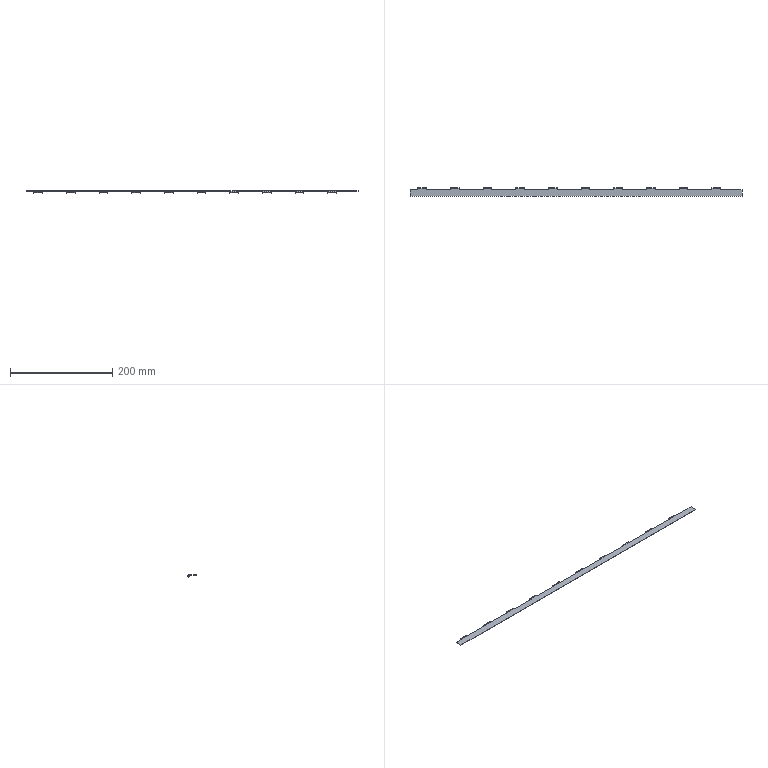Component | SolidWorks | PC-CAJ-P09-1_Bisagra de Piano 650mm-1 | 1 solid | 106 faces | volume 5204 mm3 | cylinder 60 | plane 46 | commonest cylinder face diameters 3 x30 4 x30 | material Plain Carbon Steel